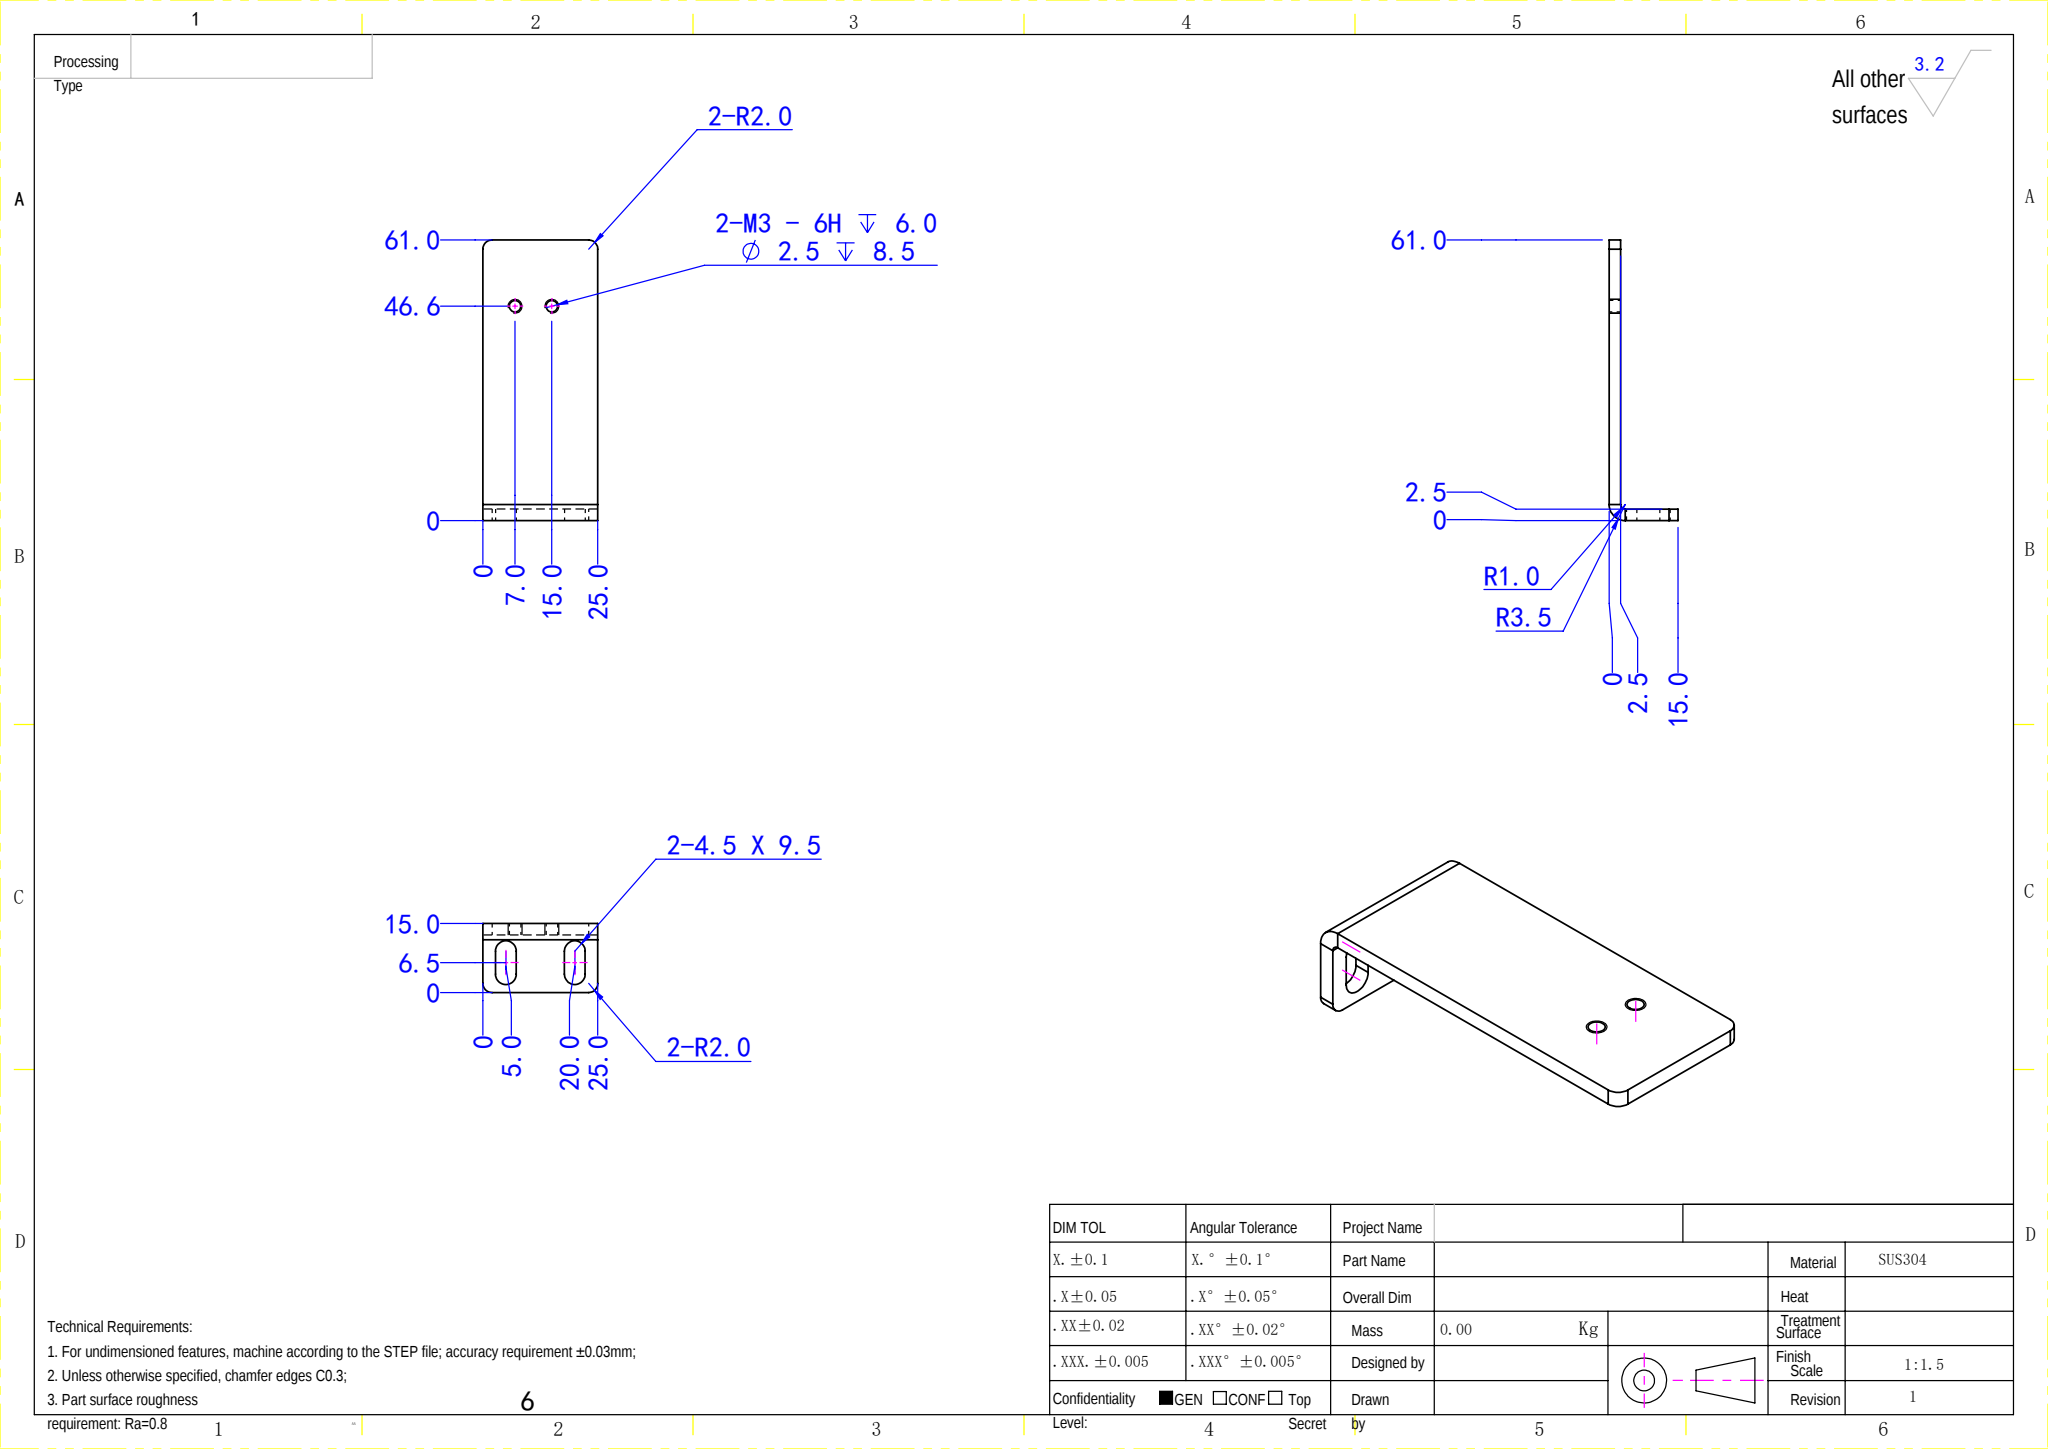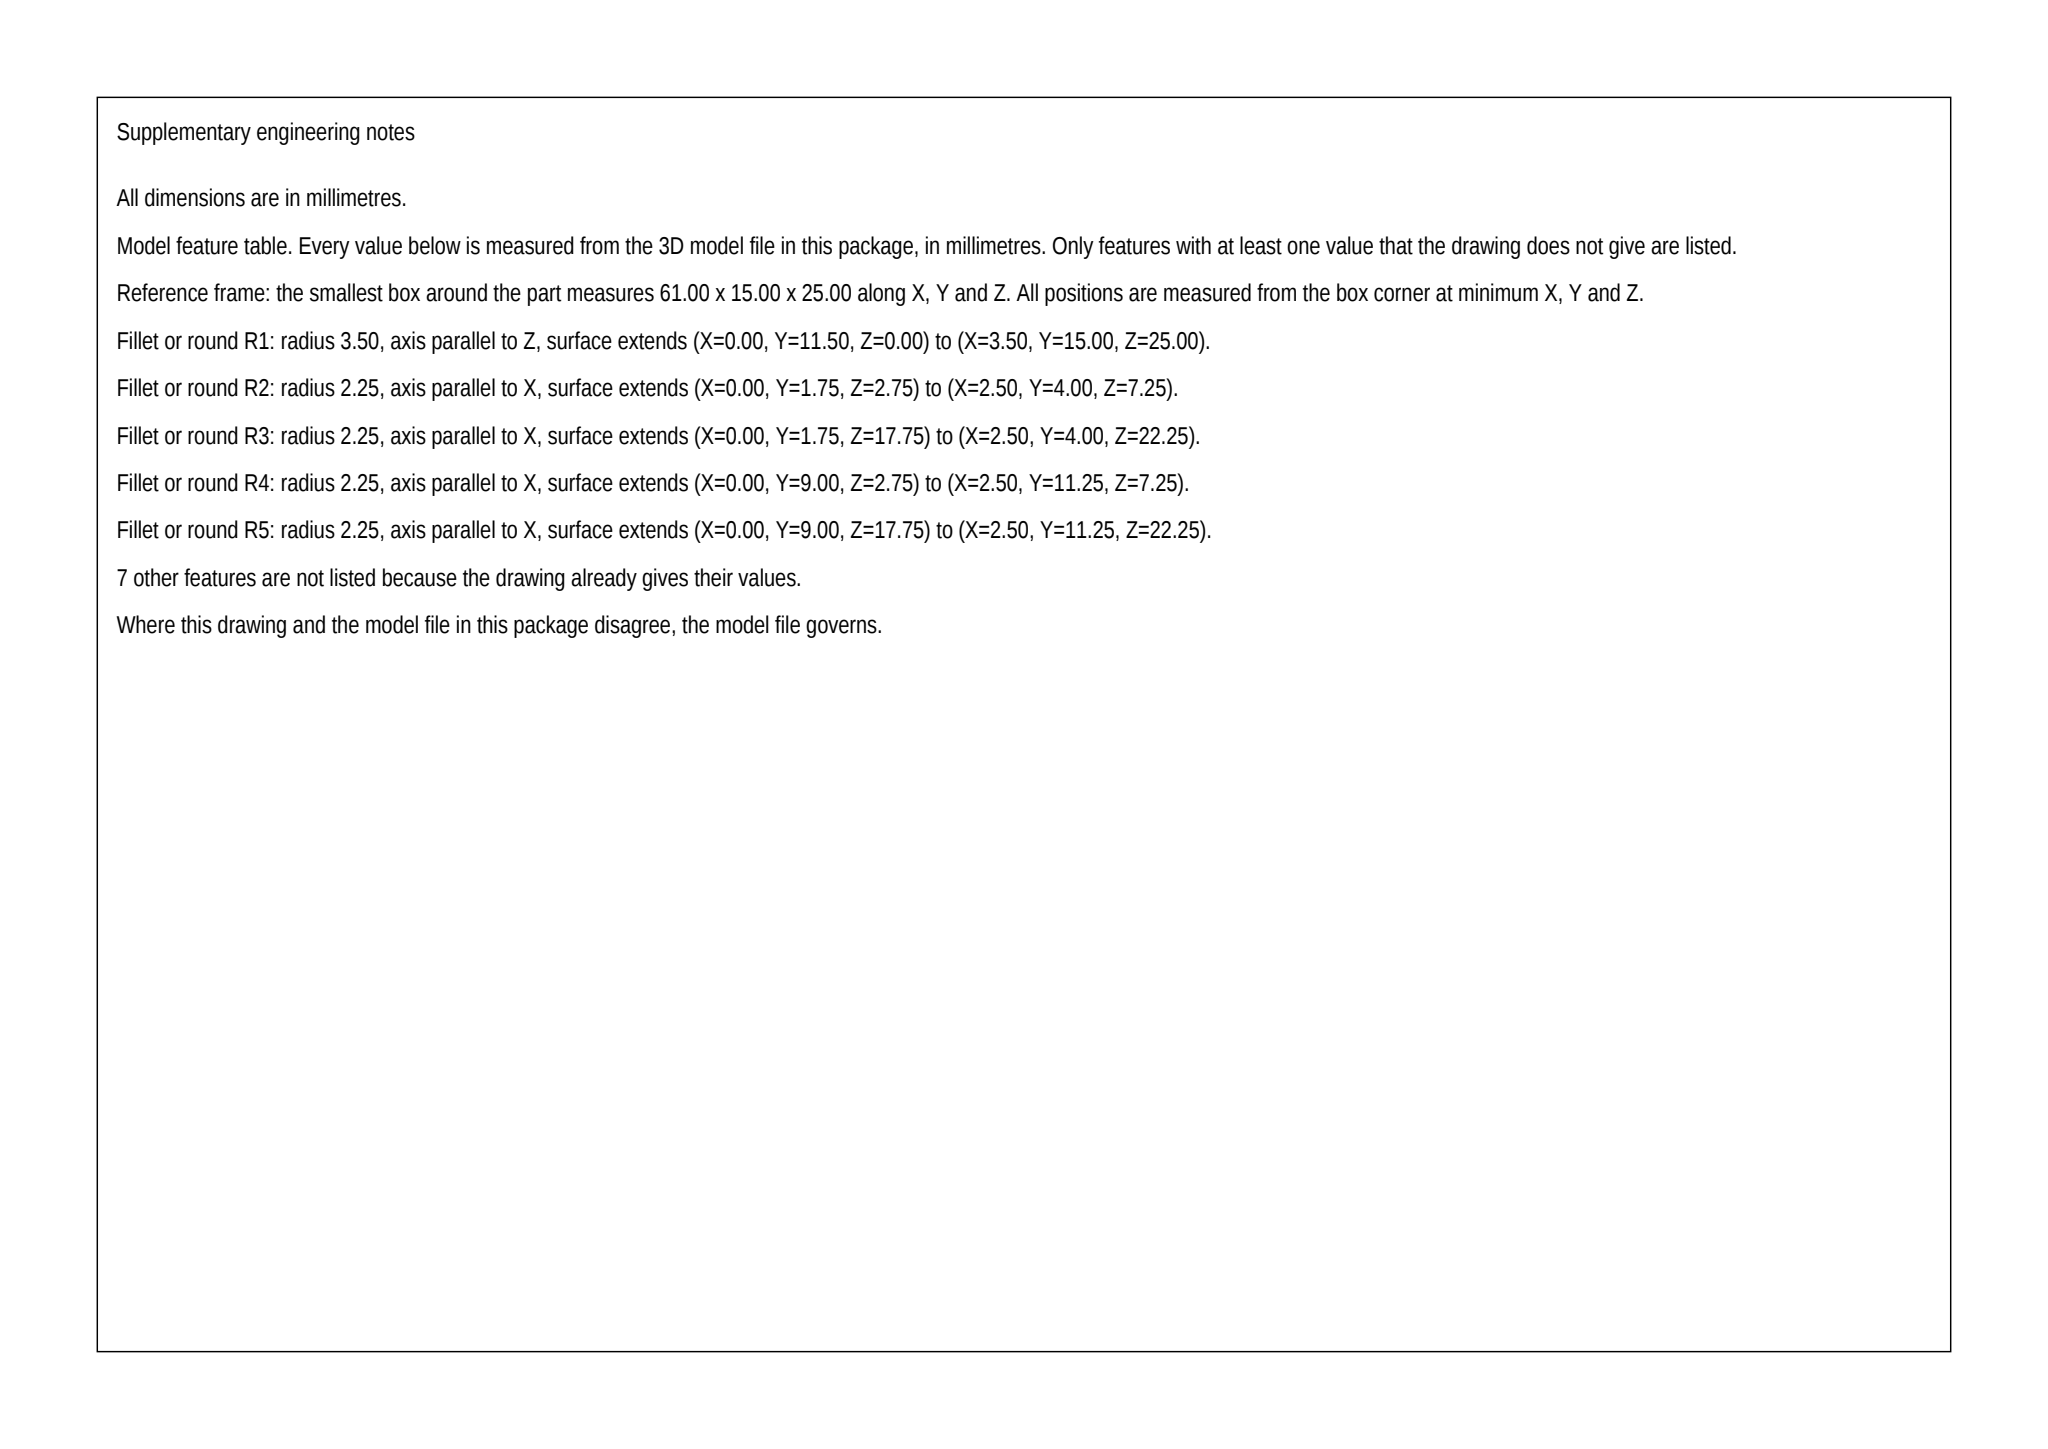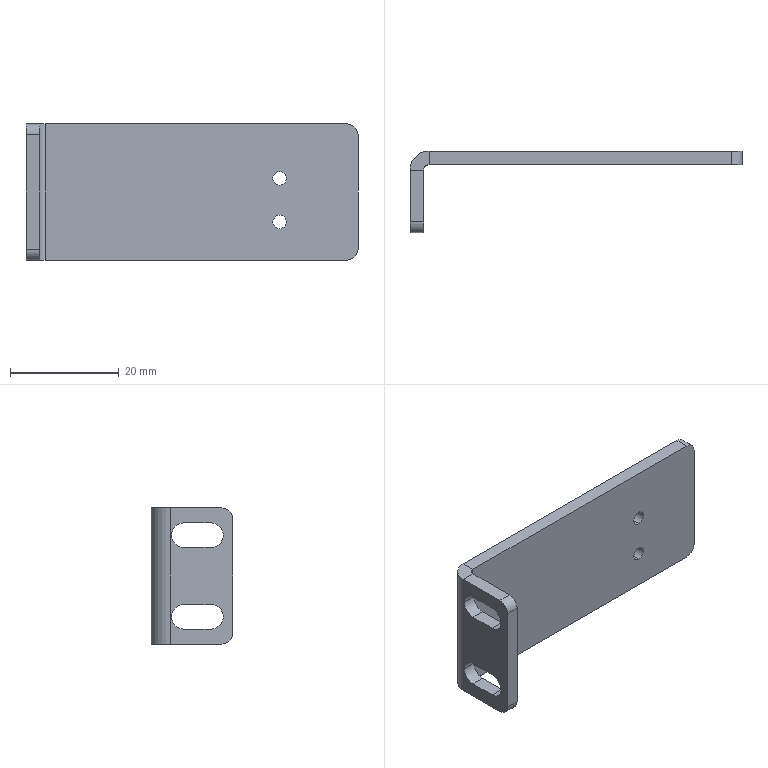Part | SolidWorks | mm | material SUS304 | 1 solid | 32 faces | box 61 x 15 x 25 mm | volume 4308 mm3 | cylinder 16 | plane 16 | commonest cylinder face diameters 4.5 x6 2.5 x4 4 x4 7 x1 2 x1